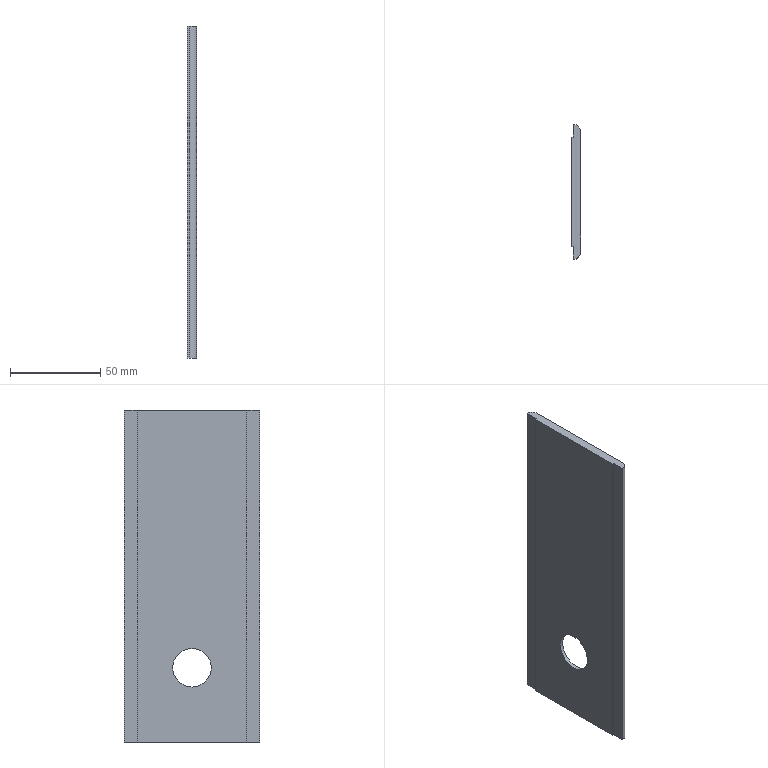Component | NX | DIGITAL_PANEL | 1 solid | 285 faces | volume 60394 mm3 | other 141 | plane 125 | cylinder 19 | commonest cylinder face diameters 8 x2 21.4 x1 42.2 x1 13.585 x1 2.199 x1 10.308 x1 2.475 x1 2.121 x1